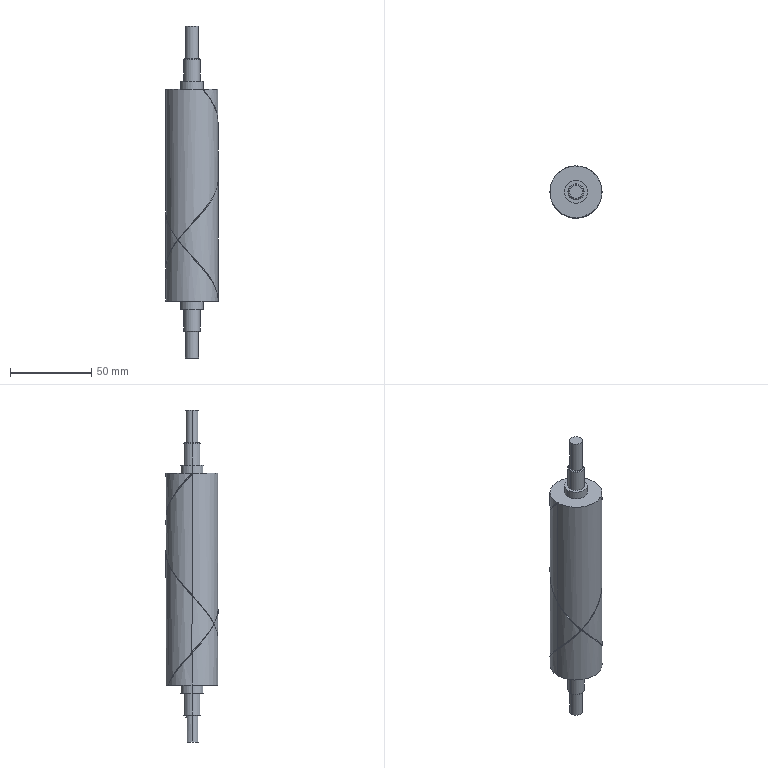Component | SolidWorks | PatternedRoller.1-1 | 1 solid | 53 faces | volume 109951 mm3 | cylinder 21 | spline 18 | plane 10 | cone 4 | commonest cylinder face diameters 32 x9 8 x4 10 x4 14 x4